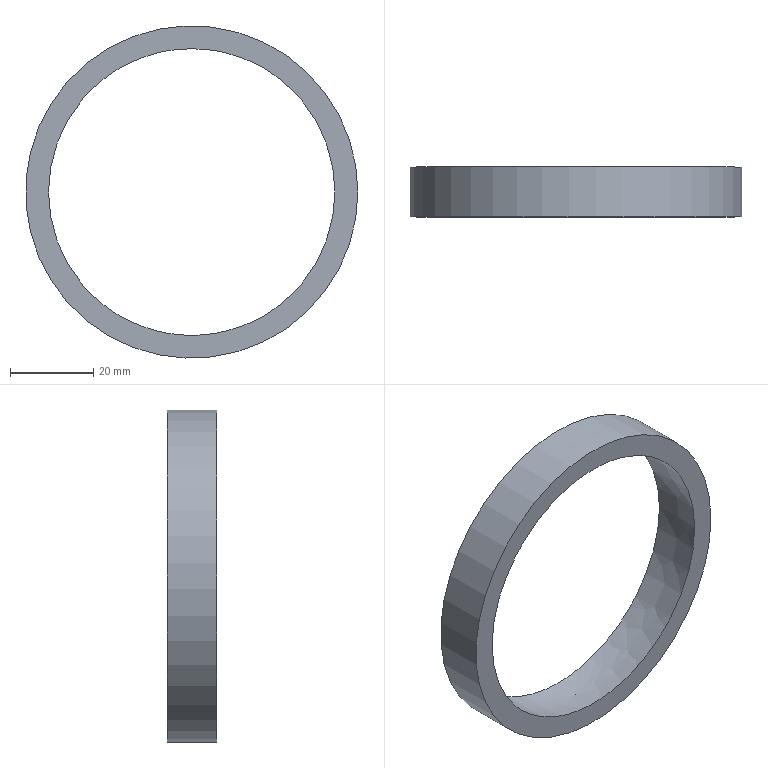Component | NX | SHIM | 1 solid | 4 faces | box 80 x 70 x 80 mm | volume 14476 mm3 | plane 2 | cylinder 1 | sphere 1 | commonest cylinder face diameters 80 x1
STEP:
#1=CARTESIAN_POINT('',(0.,0.,0.));
#2=DIRECTION('',(0.,0.,1.));
#3=DIRECTION('',(1.,0.,0.));
#4=AXIS2_PLACEMENT_3D('',#1,#2,#3);
#5=CARTESIAN_POINT('',(223.939,-6.,60.622));
#6=VERTEX_POINT('',#5);
#7=CARTESIAN_POINT('',(183.939,-6.,60.622));
#8=DIRECTION('',(0.,-1.,0.));
#9=DIRECTION('',(1.,0.,0.));
#10=AXIS2_PLACEMENT_3D('',#7,#8,#9);
#11=CIRCLE('',#10,40.);
#12=CARTESIAN_POINT('',(183.939,-6.,60.622));
#13=DIRECTION('',(0.,1.,0.));
#14=DIRECTION('',(0.,0.,1.));
#15=AXIS2_PLACEMENT_3D('',#12,#13,#14);
#16=CYLINDRICAL_SURFACE('',#15,40.);
#17=CARTESIAN_POINT('',(7.854,0.));
#18=DIRECTION('',(-1.,0.));
#19=VECTOR('',#18,1.);
#20=LINE('',#17,#19);
#21=(GEOMETRIC_REPRESENTATION_CONTEXT(2)PARAMETRIC_REPRESENTATION_CONTEXT()REPRESENTATION_CONTEXT('',''));
#22=DEFINITIONAL_REPRESENTATION('',(#20),#21);
#23=PCURVE('',#16,#22);
#24=CARTESIAN_POINT('',(183.939,-6.,60.622));
#25=DIRECTION('',(0.,-1.,0.));
#26=DIRECTION('',(0.,0.,-1.));
#27=AXIS2_PLACEMENT_3D('',#24,#25,#26);
#28=PLANE('',#27);
#29=CARTESIAN_POINT('',(0.,0.));
#30=DIRECTION('',(0.,1.));
#31=AXIS2_PLACEMENT_2D('',#29,#30);
#32=CIRCLE('',#31,40.);
#33=(GEOMETRIC_REPRESENTATION_CONTEXT(2)PARAMETRIC_REPRESENTATION_CONTEXT()REPRESENTATION_CONTEXT('',''));
#34=DEFINITIONAL_REPRESENTATION('',(#32),#33);
#35=PCURVE('',#28,#34);
#36=SURFACE_CURVE('',#11,(#23,#35),.PCURVE_S1.);
#37=EDGE_CURVE('',#6,#6,#36,.T.);
#38=ORIENTED_EDGE('',*,*,#37,.F.);
#39=CARTESIAN_POINT('',(223.939,6.,60.622));
#40=VERTEX_POINT('',#39);
#41=CARTESIAN_POINT('',(223.939,-6.,60.622));
#42=CARTESIAN_POINT('',(223.939,6.,60.622));
#43=B_SPLINE_CURVE_WITH_KNOTS('',1,(#41,#42),.UNSPECIFIED.,.F.,.F.,(2,2),(0.,12.),.PIECEWISE_BEZIER_KNOTS.);
#44=CARTESIAN_POINT('',(7.854,0.));
#45=DIRECTION('',(0.,1.));
#46=VECTOR('',#45,1.);
#47=LINE('',#44,#46);
#48=(GEOMETRIC_REPRESENTATION_CONTEXT(2)PARAMETRIC_REPRESENTATION_CONTEXT()REPRESENTATION_CONTEXT('',''));
#49=DEFINITIONAL_REPRESENTATION('',(#47),#48);
#50=PCURVE('',#16,#49);
#51=CARTESIAN_POINT('',(1.571,0.));
#52=DIRECTION('',(0.,1.));
#53=VECTOR('',#52,1.);
#54=LINE('',#51,#53);
#55=(GEOMETRIC_REPRESENTATION_CONTEXT(2)PARAMETRIC_REPRESENTATION_CONTEXT()REPRESENTATION_CONTEXT('',''));
#56=DEFINITIONAL_REPRESENTATION('',(#54),#55);
#57=PCURVE('',#16,#56);
#58=SEAM_CURVE('',#43,(#50,#57),.PCURVE_S1.);
#59=EDGE_CURVE('',#6,#40,#58,.T.);
#60=ORIENTED_EDGE('',*,*,#59,.T.);
#61=CARTESIAN_POINT('',(183.939,6.,60.622));
#62=DIRECTION('',(0.,-1.,0.));
#63=DIRECTION('',(1.,0.,0.));
#64=AXIS2_PLACEMENT_3D('',#61,#62,#63);
#65=CIRCLE('',#64,40.);
#66=CARTESIAN_POINT('',(7.854,12.));
#67=DIRECTION('',(-1.,0.));
#68=VECTOR('',#67,1.);
#69=LINE('',#66,#68);
#70=(GEOMETRIC_REPRESENTATION_CONTEXT(2)PARAMETRIC_REPRESENTATION_CONTEXT()REPRESENTATION_CONTEXT('',''));
#71=DEFINITIONAL_REPRESENTATION('',(#69),#70);
#72=PCURVE('',#16,#71);
#73=CARTESIAN_POINT('',(183.939,6.,60.622));
#74=DIRECTION('',(0.,-1.,0.));
#75=DIRECTION('',(0.,0.,-1.));
#76=AXIS2_PLACEMENT_3D('',#73,#74,#75);
#77=PLANE('',#76);
#78=CARTESIAN_POINT('',(0.,0.));
#79=DIRECTION('',(0.,1.));
#80=AXIS2_PLACEMENT_2D('',#78,#79);
#81=CIRCLE('',#80,40.);
#82=(GEOMETRIC_REPRESENTATION_CONTEXT(2)PARAMETRIC_REPRESENTATION_CONTEXT()REPRESENTATION_CONTEXT('',''));
#83=DEFINITIONAL_REPRESENTATION('',(#81),#82);
#84=PCURVE('',#77,#83);
#85=SURFACE_CURVE('',#65,(#72,#84),.PCURVE_S1.);
#86=EDGE_CURVE('',#40,#40,#85,.T.);
#87=ORIENTED_EDGE('',*,*,#86,.T.);
#88=ORIENTED_EDGE('',*,*,#59,.F.);
#89=EDGE_LOOP('',(#38,#60,#87,#88));
#90=FACE_BOUND('',#89,.T.);
#91=ADVANCED_FACE('',(#90),#16,.T.);
#92=CARTESIAN_POINT('',(183.939,-6.,26.14));
#93=VERTEX_POINT('',#92);
#94=CARTESIAN_POINT('',(183.939,-6.,60.622));
#95=DIRECTION('',(0.,-1.,0.));
#96=DIRECTION('',(0.,0.,-1.));
#97=AXIS2_PLACEMENT_3D('',#94,#95,#96);
#98=CIRCLE('',#97,34.482);
#99=CARTESIAN_POINT('',(0.,0.));
#100=DIRECTION('',(1.,0.));
#101=AXIS2_PLACEMENT_2D('',#99,#100);
#102=CIRCLE('',#101,34.482);
#103=(GEOMETRIC_REPRESENTATION_CONTEXT(2)PARAMETRIC_REPRESENTATION_CONTEXT()REPRESENTATION_CONTEXT('',''));
#104=DEFINITIONAL_REPRESENTATION('',(#102),#103);
#105=PCURVE('',#28,#104);
#106=CARTESIAN_POINT('',(183.939,-0.,60.622));
#107=DIRECTION('',(0.,0.,1.));
#108=DIRECTION('',(1.,0.,0.));
#109=AXIS2_PLACEMENT_3D('',#106,#107,#108);
#110=SPHERICAL_SURFACE('',#109,35.);
#111=CARTESIAN_POINT('',(4.712,-1.399));
#112=CARTESIAN_POINT('',(5.25,-1.372));
#113=CARTESIAN_POINT('',(5.866,-1.256));
#114=CARTESIAN_POINT('',(5.974,-0.9757));
#115=CARTESIAN_POINT('',(6.068,-0.7025));
#116=CARTESIAN_POINT('',(6.096,-0.4216));
#117=CARTESIAN_POINT('',(6.112,-0.1408));
#118=CARTESIAN_POINT('',(6.112,0.1407));
#119=CARTESIAN_POINT('',(6.095,0.4219));
#120=CARTESIAN_POINT('',(6.072,0.7016));
#121=CARTESIAN_POINT('',(5.958,0.979));
#122=CARTESIAN_POINT('',(5.927,1.244));
#123=CARTESIAN_POINT('',(4.712,1.476));
#124=CARTESIAN_POINT('',(3.497,1.244));
#125=CARTESIAN_POINT('',(3.467,0.979));
#126=CARTESIAN_POINT('',(3.353,0.7016));
#127=CARTESIAN_POINT('',(3.33,0.4219));
#128=CARTESIAN_POINT('',(3.313,0.1407));
#129=CARTESIAN_POINT('',(3.313,-0.1408));
#130=CARTESIAN_POINT('',(3.328,-0.4216));
#131=CARTESIAN_POINT('',(3.357,-0.7025));
#132=CARTESIAN_POINT('',(3.45,-0.9757));
#133=CARTESIAN_POINT('',(3.559,-1.256));
#134=CARTESIAN_POINT('',(4.175,-1.372));
#135=CARTESIAN_POINT('',(4.712,-1.399));
#136=B_SPLINE_CURVE_WITH_KNOTS('',3,(#111,#112,#113,#114,#115,#116,#117,#118,#119,#120,#121,#122,#123,#124,#125,#126,#127,#128,#129,#130,#131,#132,#133,#134,#135),.UNSPECIFIED.,.T.,.F.,(4,1,1,1,1,1,1,1,1,1,1,1,1,1,1,1,1,1,1,1,1,1,4),(0.,0.2856,0.5712,0.8568,1.142,1.428,1.714,1.999,2.285,2.57,2.856,3.142,3.427,3.713,3.998,4.284,4.57,4.855,5.141,5.426,5.712,5.998,6.283),.QUASI_UNIFORM_KNOTS.);
#137=(GEOMETRIC_REPRESENTATION_CONTEXT(2)PARAMETRIC_REPRESENTATION_CONTEXT()REPRESENTATION_CONTEXT('',''));
#138=DEFINITIONAL_REPRESENTATION('',(#136),#137);
#139=PCURVE('',#110,#138);
#140=SURFACE_CURVE('',#98,(#105,#139),.PCURVE_S1.);
#141=EDGE_CURVE('',#93,#93,#140,.T.);
#142=ORIENTED_EDGE('',*,*,#141,.F.);
#143=EDGE_LOOP('',(#142));
#144=FACE_BOUND('',#143,.T.);
#145=ORIENTED_EDGE('',*,*,#37,.T.);
#146=EDGE_LOOP('',(#145));
#147=FACE_BOUND('',#146,.T.);
#148=ADVANCED_FACE('',(#144,#147),#28,.T.);
#149=CARTESIAN_POINT('',(183.939,6.,26.14));
#150=VERTEX_POINT('',#149);
#151=CARTESIAN_POINT('',(183.939,6.,60.622));
#152=DIRECTION('',(0.,-1.,0.));
#153=DIRECTION('',(0.,0.,-1.));
#154=AXIS2_PLACEMENT_3D('',#151,#152,#153);
#155=CIRCLE('',#154,34.482);
#156=CARTESIAN_POINT('',(0.,0.));
#157=DIRECTION('',(1.,0.));
#158=AXIS2_PLACEMENT_2D('',#156,#157);
#159=CIRCLE('',#158,34.482);
#160=(GEOMETRIC_REPRESENTATION_CONTEXT(2)PARAMETRIC_REPRESENTATION_CONTEXT()REPRESENTATION_CONTEXT('',''));
#161=DEFINITIONAL_REPRESENTATION('',(#159),#160);
#162=PCURVE('',#77,#161);
#163=CARTESIAN_POINT('',(7.854,-1.399));
#164=CARTESIAN_POINT('',(7.317,-1.372));
#165=CARTESIAN_POINT('',(6.7,-1.256));
#166=CARTESIAN_POINT('',(6.592,-0.9757));
#167=CARTESIAN_POINT('',(6.499,-0.7025));
#168=CARTESIAN_POINT('',(6.47,-0.4216));
#169=CARTESIAN_POINT('',(6.455,-0.1408));
#170=CARTESIAN_POINT('',(6.454,0.1407));
#171=CARTESIAN_POINT('',(6.471,0.4219));
#172=CARTESIAN_POINT('',(6.494,0.7016));
#173=CARTESIAN_POINT('',(6.608,0.979));
#174=CARTESIAN_POINT('',(6.639,1.244));
#175=CARTESIAN_POINT('',(7.854,1.476));
#176=CARTESIAN_POINT('',(9.069,1.244));
#177=CARTESIAN_POINT('',(9.099,0.979));
#178=CARTESIAN_POINT('',(9.214,0.7016));
#179=CARTESIAN_POINT('',(9.237,0.4219));
#180=CARTESIAN_POINT('',(9.254,0.1407));
#181=CARTESIAN_POINT('',(9.253,-0.1408));
#182=CARTESIAN_POINT('',(9.238,-0.4216));
#183=CARTESIAN_POINT('',(9.209,-0.7025));
#184=CARTESIAN_POINT('',(9.116,-0.9757));
#185=CARTESIAN_POINT('',(9.008,-1.256));
#186=CARTESIAN_POINT('',(8.391,-1.372));
#187=CARTESIAN_POINT('',(7.854,-1.399));
#188=B_SPLINE_CURVE_WITH_KNOTS('',3,(#163,#164,#165,#166,#167,#168,#169,#170,#171,#172,#173,#174,#175,#176,#177,#178,#179,#180,#181,#182,#183,#184,#185,#186,#187),.UNSPECIFIED.,.T.,.F.,(4,1,1,1,1,1,1,1,1,1,1,1,1,1,1,1,1,1,1,1,1,1,4),(0.,0.2856,0.5712,0.8568,1.142,1.428,1.714,1.999,2.285,2.57,2.856,3.142,3.427,3.713,3.998,4.284,4.57,4.855,5.141,5.426,5.712,5.998,6.283),.QUASI_UNIFORM_KNOTS.);
#189=(GEOMETRIC_REPRESENTATION_CONTEXT(2)PARAMETRIC_REPRESENTATION_CONTEXT()REPRESENTATION_CONTEXT('',''));
#190=DEFINITIONAL_REPRESENTATION('',(#188),#189);
#191=PCURVE('',#110,#190);
#192=SURFACE_CURVE('',#155,(#162,#191),.PCURVE_S1.);
#193=EDGE_CURVE('',#150,#150,#192,.T.);
#194=ORIENTED_EDGE('',*,*,#193,.T.);
#195=EDGE_LOOP('',(#194));
#196=FACE_BOUND('',#195,.T.);
#197=ORIENTED_EDGE('',*,*,#86,.F.);
#198=EDGE_LOOP('',(#197));
#199=FACE_BOUND('',#198,.T.);
#200=ADVANCED_FACE('',(#196,#199),#77,.F.);
#201=ORIENTED_EDGE('',*,*,#141,.F.);
#202=EDGE_LOOP('',(#201));
#203=FACE_BOUND('',#202,.F.);
#204=ORIENTED_EDGE('',*,*,#193,.T.);
#205=EDGE_LOOP('',(#204));
#206=FACE_BOUND('',#205,.F.);
#207=CARTESIAN_POINT('',(183.939,-0.,25.622));
#208=VERTEX_POINT('',#207);
#209=VERTEX_LOOP('',#208);
#210=FACE_BOUND('',#209,.F.);
#211=ADVANCED_FACE('',(#203,#206,#210),#110,.F.);
#212=CLOSED_SHELL('',(#91,#148,#200,#211));
#213=MANIFOLD_SOLID_BREP('',#212);
#214=(LENGTH_UNIT()NAMED_UNIT(*)SI_UNIT(.MILLI.,.METRE.));
#215=UNCERTAINTY_MEASURE_WITH_UNIT(LENGTH_MEASURE(0.000005),#214,'','');
#216=(NAMED_UNIT(*)PLANE_ANGLE_UNIT()SI_UNIT($,.RADIAN.));
#217=(NAMED_UNIT(*)SI_UNIT($,.STERADIAN.)SOLID_ANGLE_UNIT());
#218=(GEOMETRIC_REPRESENTATION_CONTEXT(3)GLOBAL_UNCERTAINTY_ASSIGNED_CONTEXT((#215))GLOBAL_UNIT_ASSIGNED_CONTEXT((#214,#216,#217))REPRESENTATION_CONTEXT('',''));
#219=ADVANCED_BREP_SHAPE_REPRESENTATION('',(#4,#213),#218);